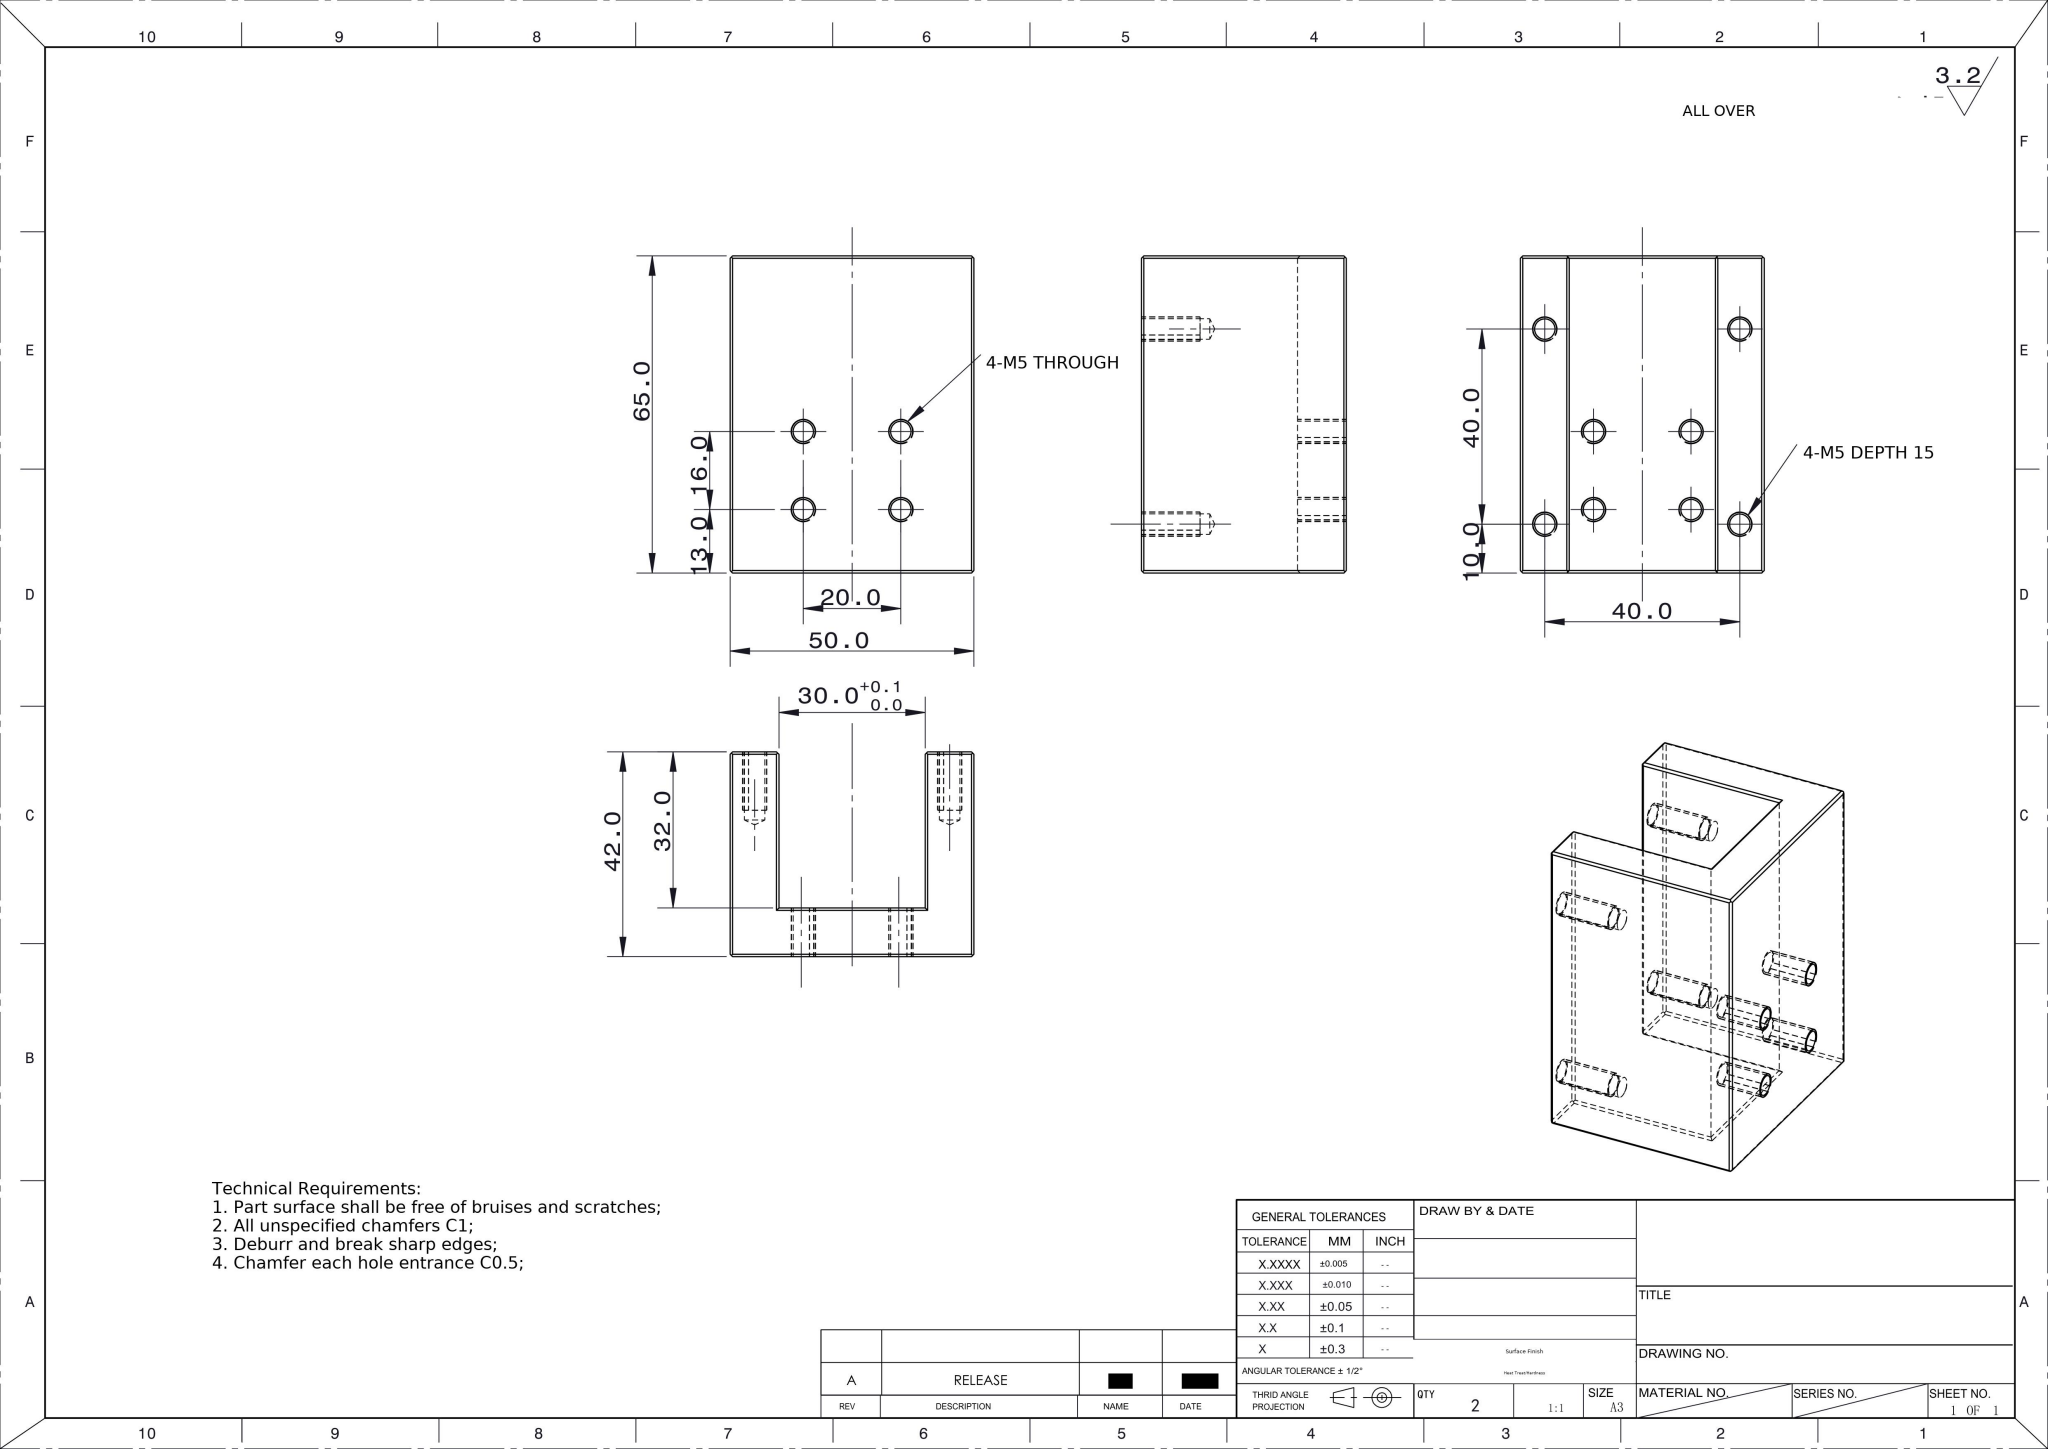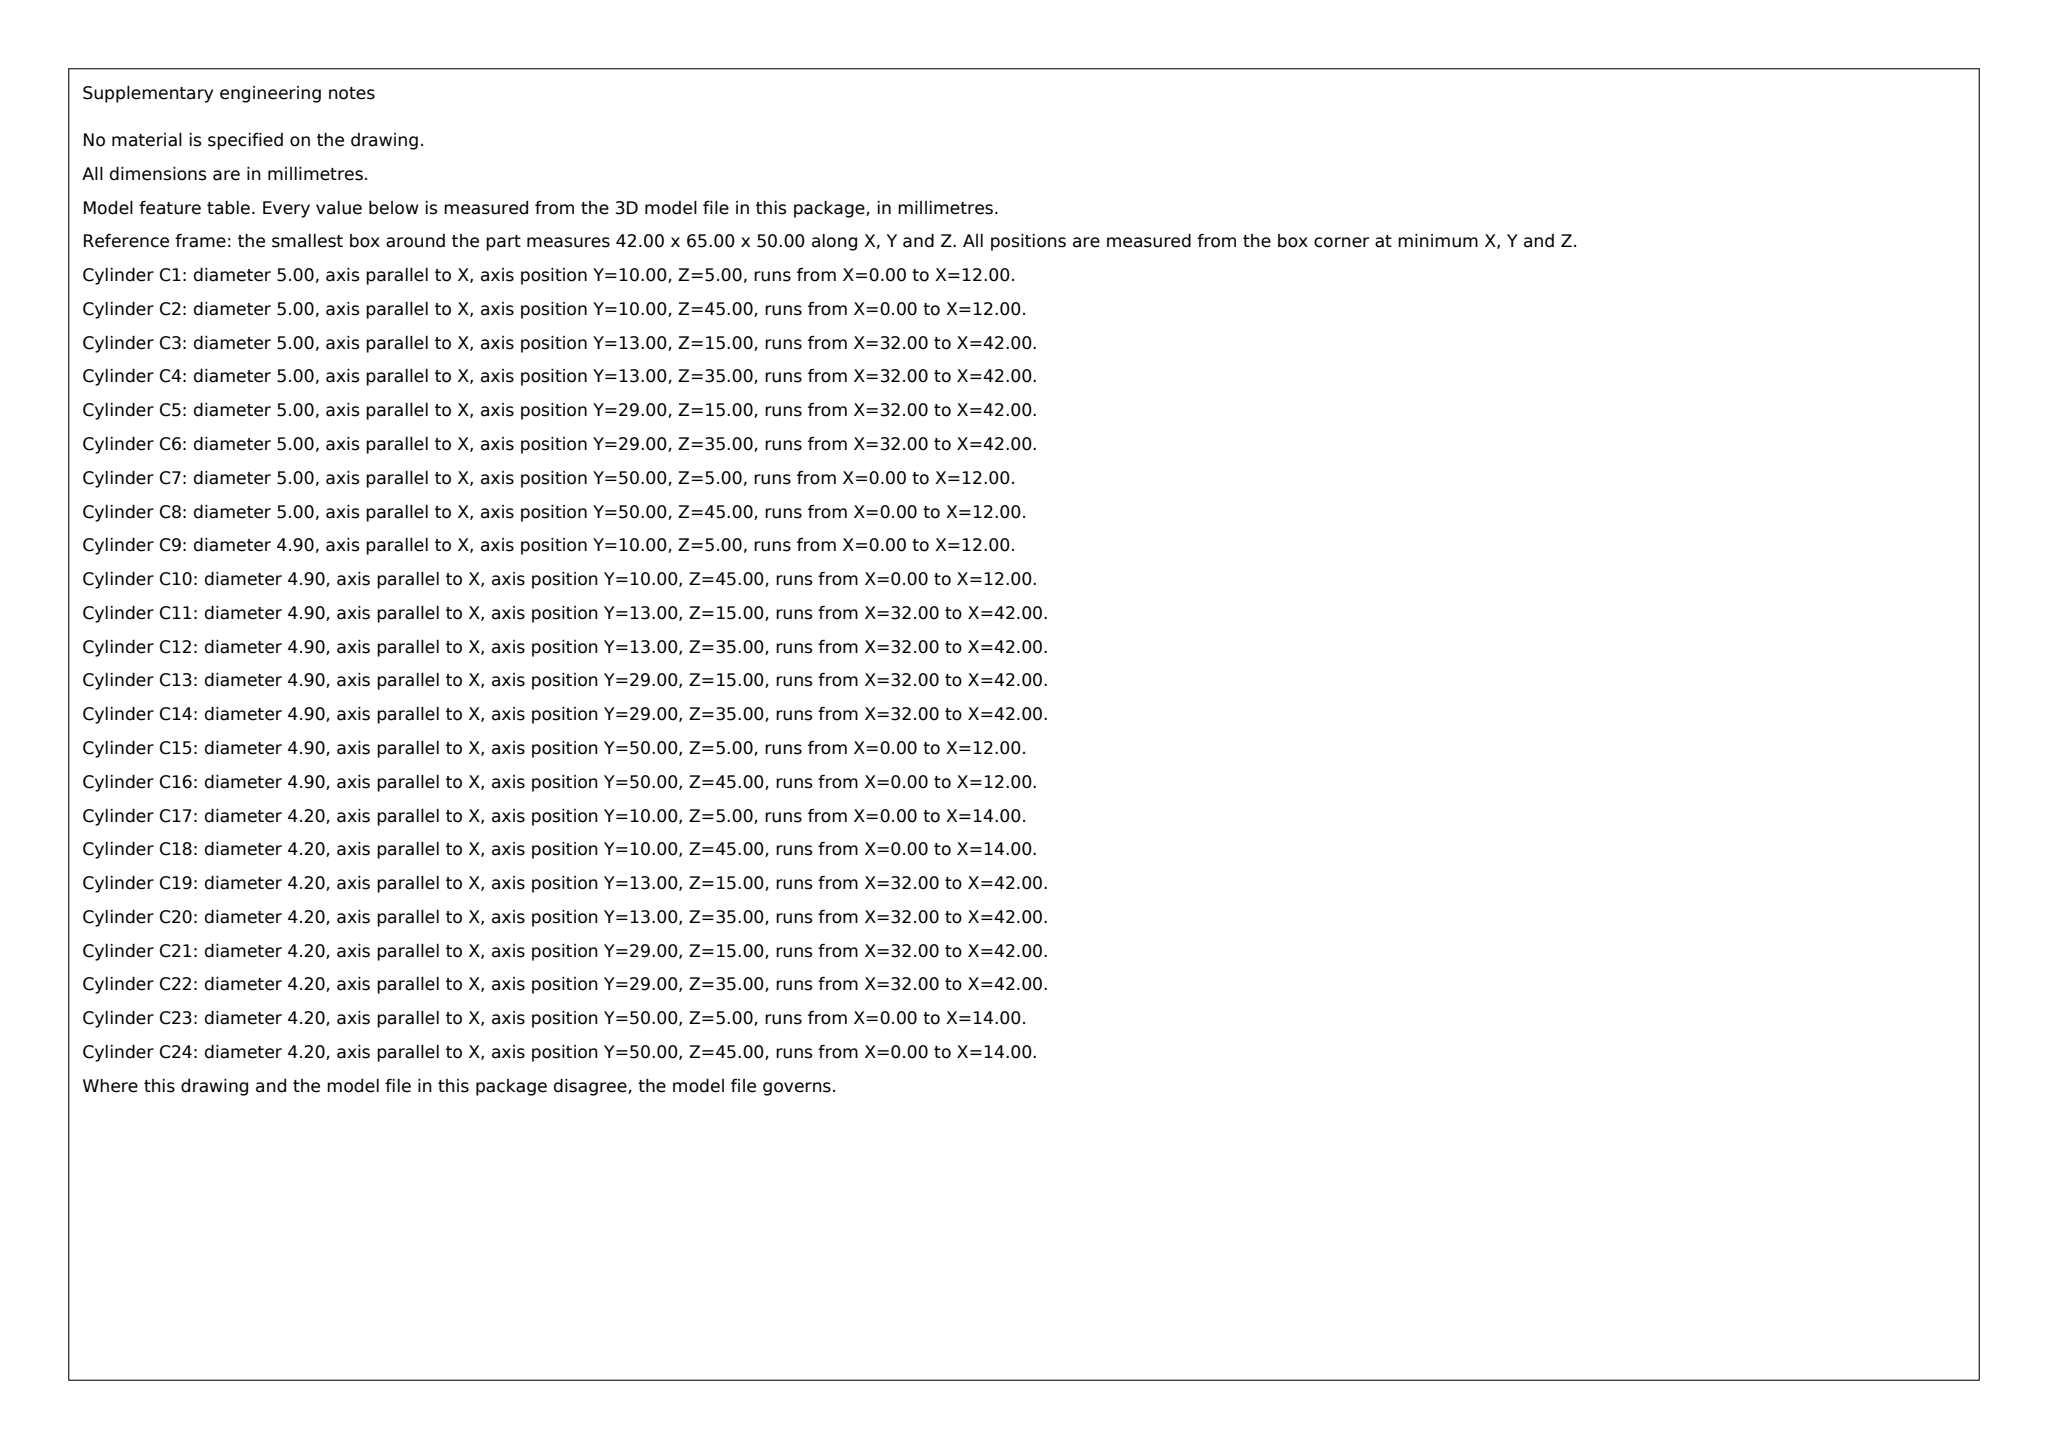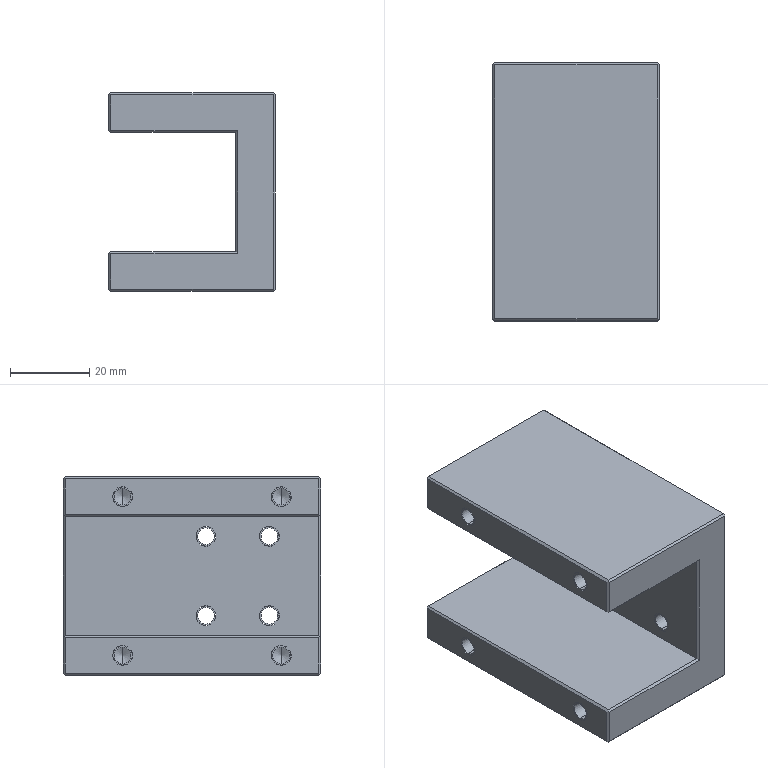Part | SolidWorks | mm | 1 solid | 132 faces | box 42 x 65 x 50 mm | volume 72579 mm3 | cylinder 68 | plane 56 | cone 8 | commonest cylinder face diameters 4.9 x24 4.2 x24 5 x20